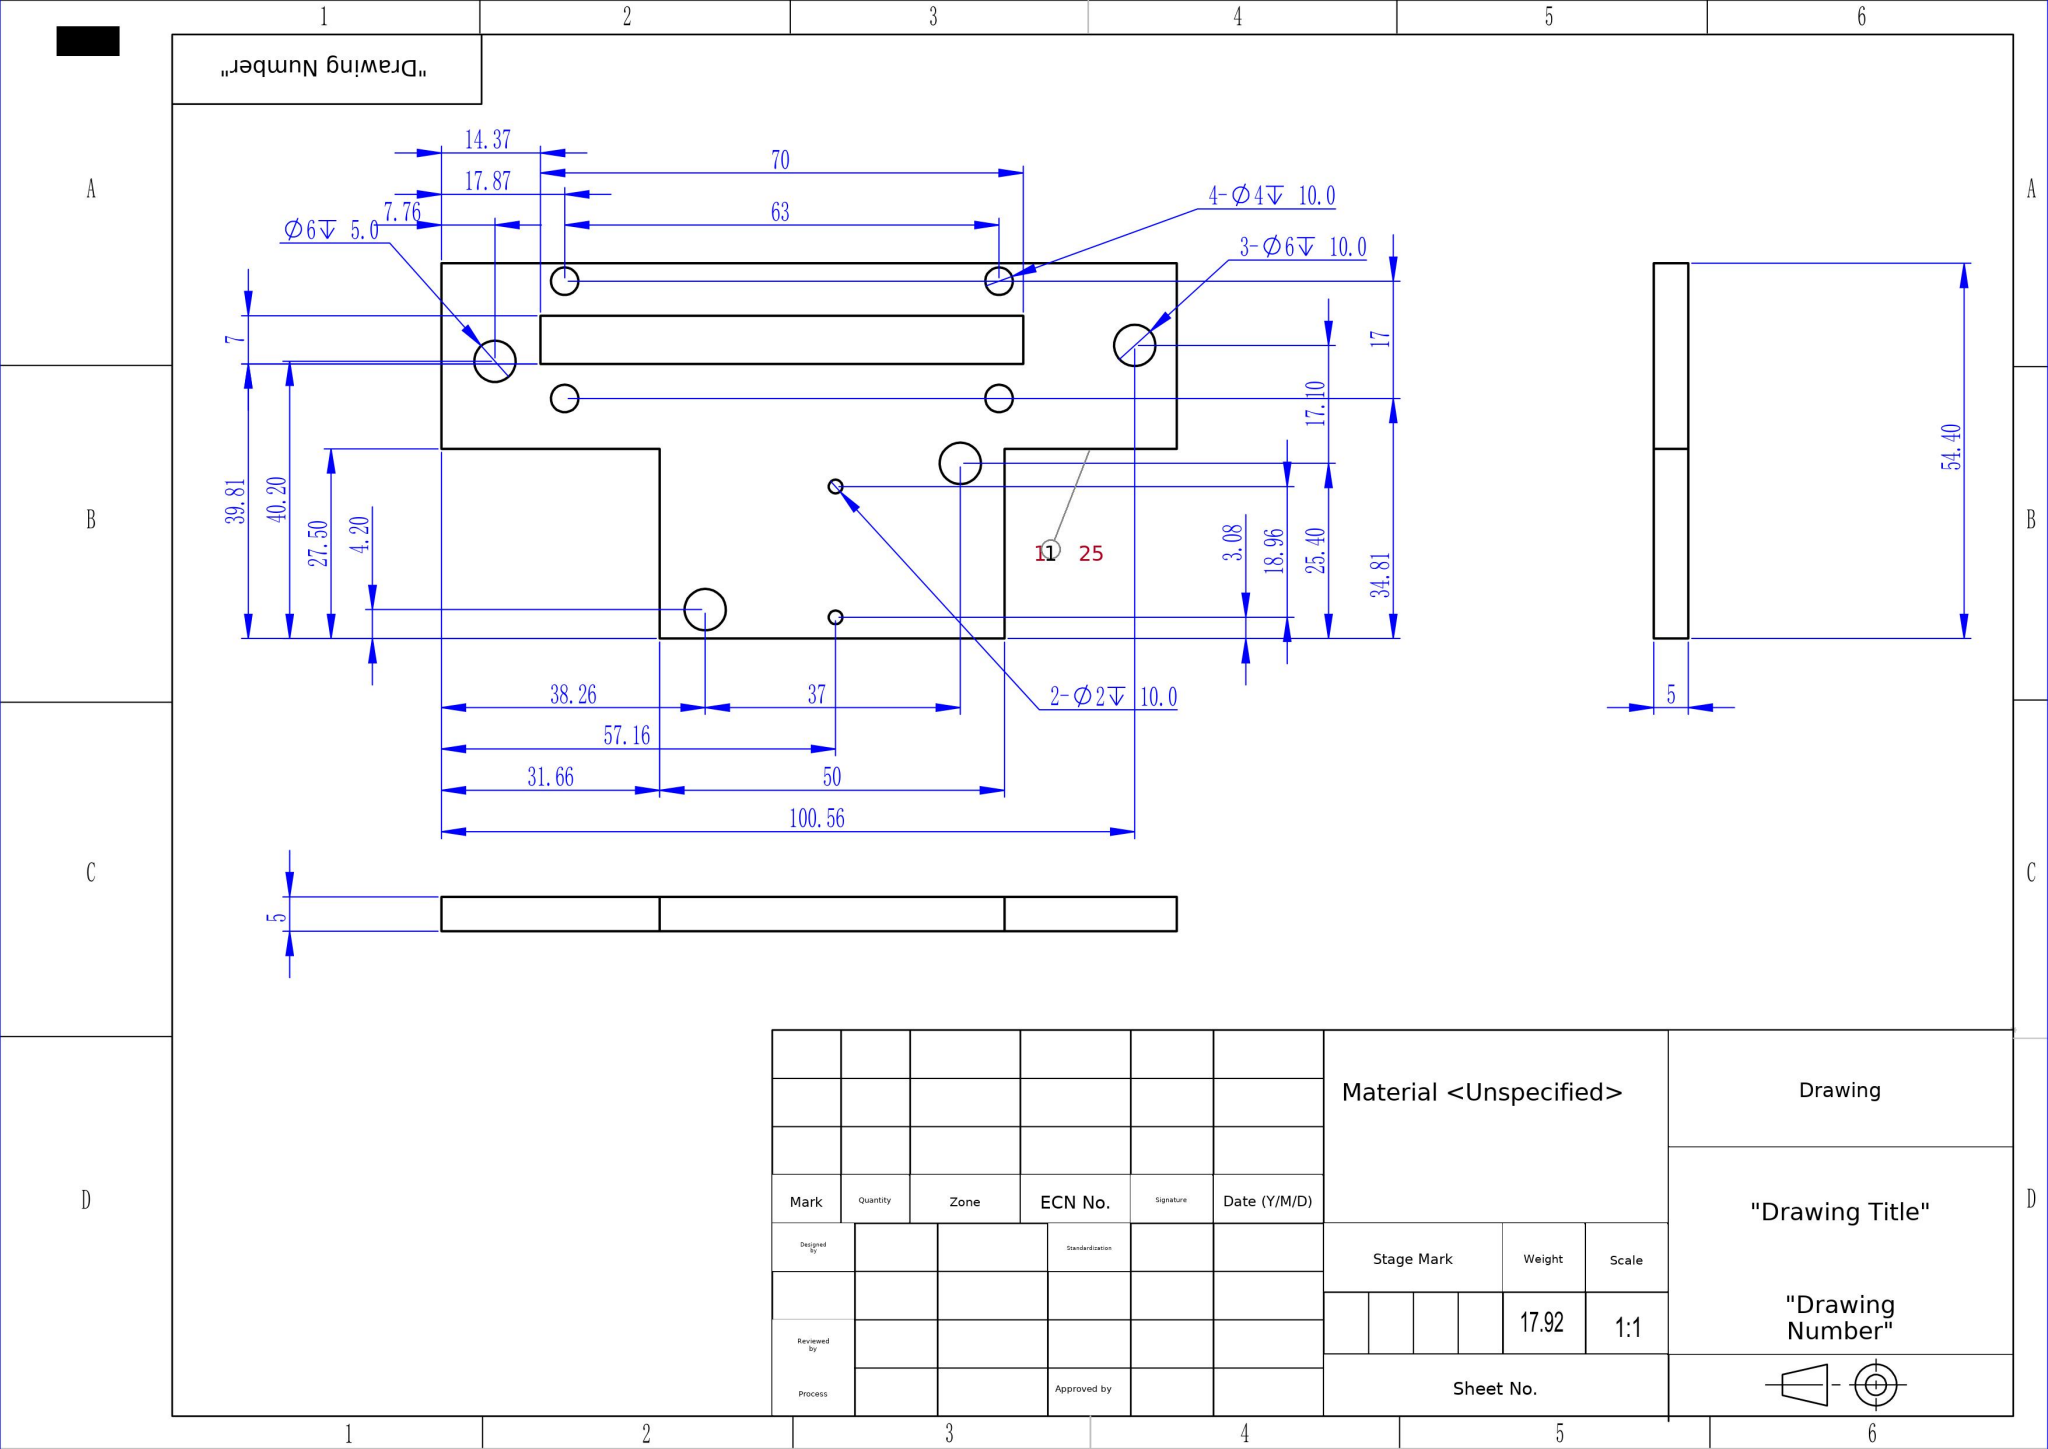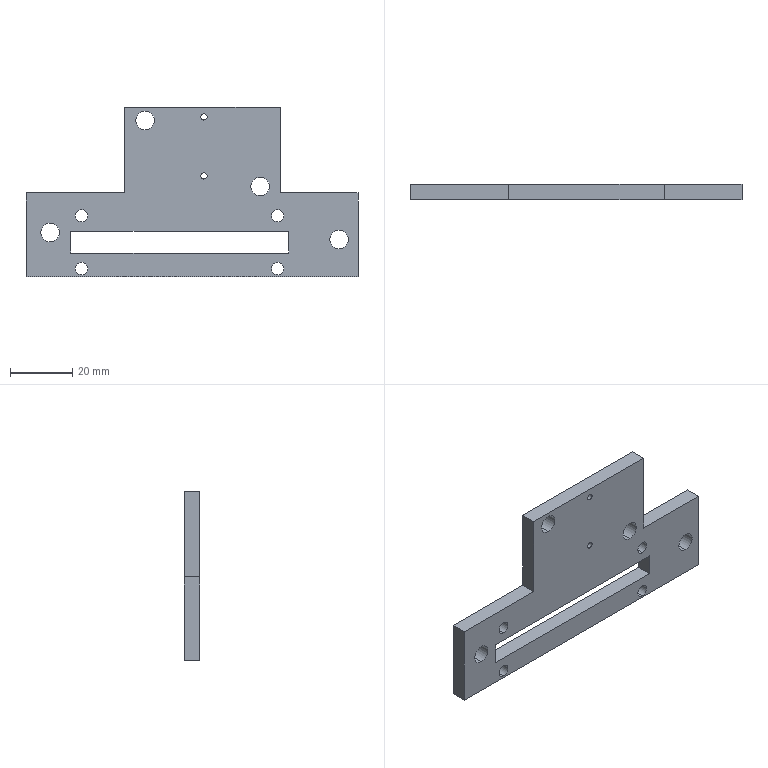Part | SolidWorks | mm | 1 solid | 34 faces | box 106.66 x 5 x 54.4 mm | volume 17921 mm3 | cylinder 20 | plane 14 | commonest cylinder face diameters 4 x8 6 x8 2 x4
build123d program:
from build123d import *

# Parameters (mm, degrees)
SKETCH1_W           = 50
SKETCH1_H           = 40
BOSS_EXTRUDE1_DEPTH = 5
SKETCH2_W           = 100
SKETCH2_H           = 25
BOSS_EXTRUDE2_DEPTH = 5
SKETCH3_R           = 3
CUT_EXTRUDE1_DEPTH  = 10
SKETCH4_R           = 1
CUT_EXTRUDE2_DEPTH  = 10
SKETCH5_W           = 100
SKETCH5_H           = 16.902
BOSS_EXTRUDE3_DEPTH = 5
SKETCH6_W           = 3.34
SKETCH6_H           = 41.902
CUT_EXTRUDE3_DEPTH  = 10
SKETCH9_W           = 10
SKETCH9_H           = 41.902
BOSS_EXTRUDE4_DEPTH = 5
SKETCH10_R          = 3
CUT_EXTRUDE4_DEPTH  = 5
SKETCH11_W          = 106.66
SKETCH11_H          = 15.005
CUT_EXTRUDE5_DEPTH  = 5
SKETCH12_R          = 2
SKETCH12_W          = 70
SKETCH12_H          = 7
CUT_EXTRUDE6_DEPTH  = 10


with BuildPart() as part:
    # Sketch1 → Boss-Extrude1 (new body)
    with BuildSketch(Plane(origin=(0, 0, 0), x_dir=(1, 0, 0), z_dir=(0, 1, 0))):
        with Locations((25, 20)):
            Rectangle(SKETCH1_W, SKETCH1_H)
    extrude(amount=BOSS_EXTRUDE1_DEPTH)

    # Sketch2 → Boss-Extrude2 (add)
    with BuildSketch(Plane(origin=(0, 5, 0), x_dir=(1, 0, 0), z_dir=(0, 1, 0))):
        with Locations((25, 40)):
            Rectangle(SKETCH2_W, SKETCH2_H)
    extrude(amount=-BOSS_EXTRUDE2_DEPTH)

    # Sketch3 → Cut-Extrude1 (cut)
    with BuildSketch(Plane.XZ):
        with Locations(Location((6.6, -4.2, 0), (0, 0, 270))):
            Circle(SKETCH3_R)
        with Locations(Location((43.6, -25.4, 0), (0, 0, 270))):
            Circle(SKETCH3_R)
        with Locations(Location((68.9, -42.5, 0), (0, 0, 270))):
            Circle(SKETCH3_R)
    extrude(amount=-CUT_EXTRUDE1_DEPTH, mode=Mode.SUBTRACT)

    # Sketch4 → Cut-Extrude2 (cut)
    with BuildSketch(Plane.XZ):
        with Locations(Location((25.5, -3.08, 0), (0, 0, 270))):
            Circle(SKETCH4_R)
        with Locations(Location((25.5, -22.04, 0), (0, 0, 270))):
            Circle(SKETCH4_R)
    extrude(amount=-CUT_EXTRUDE2_DEPTH, mode=Mode.SUBTRACT)

    # Sketch5 → Boss-Extrude3 (add)
    with BuildSketch(Plane.XZ):
        with Locations((25, -60.951)):
            Rectangle(SKETCH5_W, SKETCH5_H)
    extrude(amount=-BOSS_EXTRUDE3_DEPTH)

    # Sketch6 → Cut-Extrude3 (cut)
    with BuildSketch(Plane.XZ):
        with Locations((-23.33, -48.451)):
            Rectangle(SKETCH6_W, SKETCH6_H)
    extrude(amount=-CUT_EXTRUDE3_DEPTH, mode=Mode.SUBTRACT)

    # Sketch9 → Boss-Extrude4 (add)
    with BuildSketch(Plane.XZ):
        with Locations((-26.66, -48.451)):
            Rectangle(SKETCH9_W, SKETCH9_H)
    extrude(amount=-BOSS_EXTRUDE4_DEPTH)

    # Sketch10 → Cut-Extrude4 (cut)
    with BuildSketch(Plane.XZ):
        with Locations(Location((-23.9, -40.2, 0), (0, 0, 270))):
            Circle(SKETCH10_R)
    extrude(amount=-CUT_EXTRUDE4_DEPTH, mode=Mode.SUBTRACT)

    # Sketch11 → Cut-Extrude5 (cut)
    with BuildSketch(Plane.XZ):
        with Locations((21.67, -61.9)):
            Rectangle(SKETCH11_W, SKETCH11_H)
    extrude(amount=-CUT_EXTRUDE5_DEPTH, mode=Mode.SUBTRACT)

    # Sketch12 → Cut-Extrude6 (cut)
    with BuildSketch(Plane.XZ):
        with Locations(Location((-13.786, -34.809, 0), (0, 0, 270))):
            Circle(SKETCH12_R)
        with Locations(Location((49.214, -34.809, 0), (0, 0, 270))):
            Circle(SKETCH12_R)
        with Locations(Location((-13.786, -51.809, 0), (0, 0, 270))):
            Circle(SKETCH12_R)
        with Locations(Location((49.214, -51.809, 0), (0, 0, 270))):
            Circle(SKETCH12_R)
        with Locations((17.714, -43.309)):
            Rectangle(SKETCH12_W, SKETCH12_H)
    extrude(amount=-CUT_EXTRUDE6_DEPTH, mode=Mode.SUBTRACT)


solid = part.part